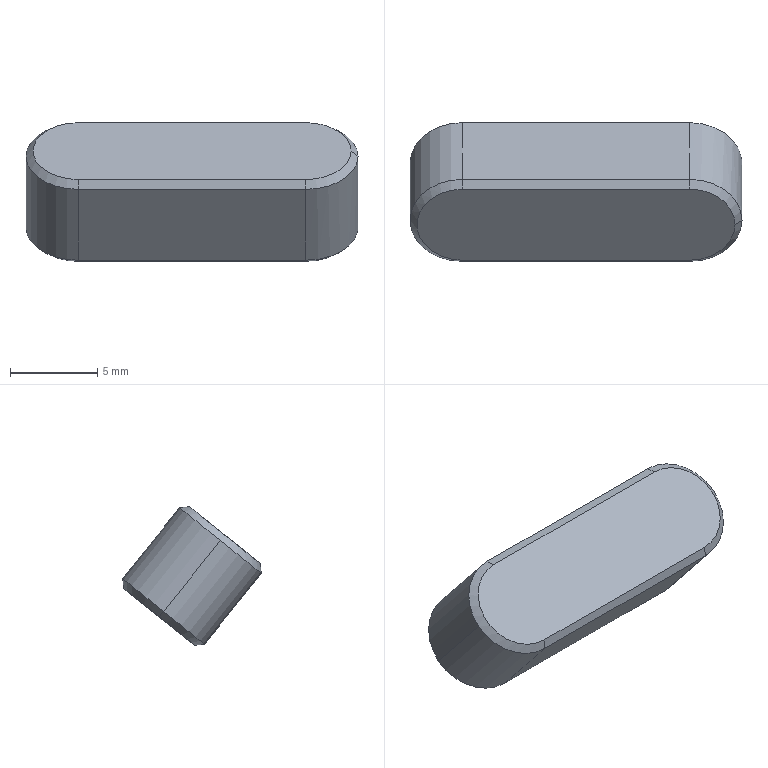Component | SolidWorks | Key6-6-25-2 | 1 solid | 17 faces | box 19 x 7.93 x 7.93 mm | volume 631 mm3 | plane 8 | cone 6 | cylinder 3 | commonest cylinder face diameters 6 x3
build123d program:
from build123d import *

# Parameters (mm, degrees)
BOSS_EXTRUDE1_DEPTH = 6
CHAMFER1_SIZE2      = 0.4
CHAMFER1_SIZE       = 0.4


with BuildPart() as part:
    # Sketch1 → Boss-Extrude1 (new body)
    with BuildSketch(Plane(origin=(0, 0, 4), x_dir=(1, 0, 0), z_dir=(0, -1, 0))):
        with BuildLine():
            Line((-3, 9), (-3, -4))
            ThreePointArc((-3, -4), (0, -7), (3, -4))
            Line((3, -4), (3, 9))
            ThreePointArc((3, 9), (0, 12), (-3, 9))
        make_face()
    extrude(amount=-BOSS_EXTRUDE1_DEPTH)

    # Chamfer1
    chamfer1_edges = [part.edges().sort_by_distance(p)[0] for p in [
        (0, 6, -3),
        (3, 6, 6.5),
        (0, 6, 16),
        (3, 0, 6.5),
        (0, 0, -3),
        (-3, 0, 6.5),
        (0, 0, 16),
        (-3, 6, 6.5),
    ]]
    chamfer(chamfer1_edges, length=CHAMFER1_SIZE, length2=CHAMFER1_SIZE2)


solid = part.part

# Placed as in the assembly
solid = solid.moved(Location((-531.299, 8.129, -10.145), (128.707, -90, 0)))
STEP:
#1=COLOUR_RGB('',0.7922,0.8196,0.9333);
#2=FILL_AREA_STYLE_COLOUR('',#1);
#3=FILL_AREA_STYLE('',(#2));
#4=SURFACE_STYLE_FILL_AREA(#3);
#5=SURFACE_SIDE_STYLE('',(#4));
#6=SURFACE_STYLE_USAGE(.BOTH.,#5);
#7=PRESENTATION_STYLE_ASSIGNMENT((#6));
#8=CARTESIAN_POINT('',(-21.531,0.3201,-0.3994));
#9=VERTEX_POINT('',#8);
#10=CARTESIAN_POINT('',(-21.429,0.3999,-0.3354));
#11=VERTEX_POINT('',#10);
#12=CARTESIAN_POINT('',(-21.429,0.3201,-0.3994));
#13=DIRECTION('',(-0.,0.6253,-0.7803));
#14=DIRECTION('',(-1.,-0.,-0.));
#15=AXIS2_PLACEMENT_3D('',#12,#13,#14);
#16=CIRCLE('',#15,0.1024);
#17=EDGE_CURVE('',#9,#11,#16,.T.);
#18=ORIENTED_EDGE('',*,*,#17,.F.);
#19=CARTESIAN_POINT('',(-21.547,0.3102,-0.3871));
#20=VERTEX_POINT('',#19);
#21=CARTESIAN_POINT('',(-21.547,0.3102,-0.3871));
#22=DIRECTION('',(-0.7071,-0.4422,0.5518));
#23=VECTOR('',#22,39.37);
#24=LINE('',#21,#23);
#25=EDGE_CURVE('',#9,#20,#24,.T.);
#26=ORIENTED_EDGE('',*,*,#25,.T.);
#27=CARTESIAN_POINT('',(-21.429,0.4024,-0.3132));
#28=VERTEX_POINT('',#27);
#29=CARTESIAN_POINT('',(-21.429,0.3102,-0.3871));
#30=DIRECTION('',(0.,-0.6253,0.7803));
#31=DIRECTION('',(-1.,-0.,-0.));
#32=AXIS2_PLACEMENT_3D('',#29,#30,#31);
#33=CIRCLE('',#32,0.1181);
#34=EDGE_CURVE('',#28,#20,#33,.T.);
#35=ORIENTED_EDGE('',*,*,#34,.F.);
#36=CARTESIAN_POINT('',(-21.429,0.3999,-0.3354));
#37=DIRECTION('',(-0.,0.1096,0.994));
#38=VECTOR('',#37,39.37);
#39=LINE('',#36,#38);
#40=EDGE_CURVE('',#11,#28,#39,.T.);
#41=ORIENTED_EDGE('',*,*,#40,.F.);
#42=EDGE_LOOP('',(#18,#26,#35,#41));
#43=FACE_OUTER_BOUND('',#42,.T.);
#44=CARTESIAN_POINT('',(-21.429,0.3102,-0.3871));
#45=DIRECTION('',(0.,-0.6253,0.7803));
#46=DIRECTION('',(-1.,-0.,-0.));
#47=AXIS2_PLACEMENT_3D('',#44,#45,#46);
#48=CONICAL_SURFACE('',#47,0.1181,0.7854);
#49=ADVANCED_FACE('',(#43),#48,.T.);
#50=CARTESIAN_POINT('',(-20.815,0.1723,-0.2151));
#51=VERTEX_POINT('',#50);
#52=CARTESIAN_POINT('',(-20.917,0.2522,-0.151));
#53=VERTEX_POINT('',#52);
#54=CARTESIAN_POINT('',(-20.917,0.1723,-0.2151));
#55=DIRECTION('',(0.,-0.6253,0.7803));
#56=DIRECTION('',(-1.,-0.,-0.));
#57=AXIS2_PLACEMENT_3D('',#54,#55,#56);
#58=CIRCLE('',#57,0.1024);
#59=EDGE_CURVE('',#51,#53,#58,.T.);
#60=ORIENTED_EDGE('',*,*,#59,.F.);
#61=CARTESIAN_POINT('',(-20.799,0.1822,-0.2273));
#62=VERTEX_POINT('',#61);
#63=CARTESIAN_POINT('',(-20.815,0.1723,-0.2151));
#64=DIRECTION('',(0.7071,0.4422,-0.5518));
#65=VECTOR('',#64,39.37);
#66=LINE('',#63,#65);
#67=EDGE_CURVE('',#51,#62,#66,.T.);
#68=ORIENTED_EDGE('',*,*,#67,.T.);
#69=CARTESIAN_POINT('',(-20.917,0.2744,-0.1535));
#70=VERTEX_POINT('',#69);
#71=CARTESIAN_POINT('',(-20.917,0.1822,-0.2273));
#72=DIRECTION('',(-0.,0.6253,-0.7803));
#73=DIRECTION('',(-1.,-0.,-0.));
#74=AXIS2_PLACEMENT_3D('',#71,#72,#73);
#75=CIRCLE('',#74,0.1181);
#76=EDGE_CURVE('',#70,#62,#75,.T.);
#77=ORIENTED_EDGE('',*,*,#76,.F.);
#78=CARTESIAN_POINT('',(-20.917,0.2744,-0.1535));
#79=DIRECTION('',(0.,-0.994,0.1096));
#80=VECTOR('',#79,39.37);
#81=LINE('',#78,#80);
#82=EDGE_CURVE('',#70,#53,#81,.T.);
#83=ORIENTED_EDGE('',*,*,#82,.T.);
#84=EDGE_LOOP('',(#60,#68,#77,#83));
#85=FACE_OUTER_BOUND('',#84,.T.);
#86=CARTESIAN_POINT('',(-20.917,0.1723,-0.2151));
#87=DIRECTION('',(-0.,0.6253,-0.7803));
#88=DIRECTION('',(1.,0.,0.));
#89=AXIS2_PLACEMENT_3D('',#86,#87,#88);
#90=CONICAL_SURFACE('',#89,0.1024,0.7854);
#91=ADVANCED_FACE('',(#85),#90,.T.);
#92=ORIENTED_EDGE('',*,*,#34,.T.);
#93=CARTESIAN_POINT('',(-21.547,0.1822,-0.2273));
#94=VERTEX_POINT('',#93);
#95=CARTESIAN_POINT('',(-21.547,0.3201,-0.3994));
#96=DIRECTION('',(0.,-0.6253,0.7803));
#97=VECTOR('',#96,39.37);
#98=LINE('',#95,#97);
#99=EDGE_CURVE('',#20,#94,#98,.T.);
#100=ORIENTED_EDGE('',*,*,#99,.T.);
#101=CARTESIAN_POINT('',(-21.429,0.2744,-0.1535));
#102=VERTEX_POINT('',#101);
#103=CARTESIAN_POINT('',(-21.429,0.1822,-0.2273));
#104=DIRECTION('',(-0.,0.6253,-0.7803));
#105=DIRECTION('',(-1.,-0.,-0.));
#106=AXIS2_PLACEMENT_3D('',#103,#104,#105);
#107=CIRCLE('',#106,0.1181);
#108=EDGE_CURVE('',#94,#102,#107,.T.);
#109=ORIENTED_EDGE('',*,*,#108,.T.);
#110=CARTESIAN_POINT('',(-21.429,0.4122,-0.3255));
#111=DIRECTION('',(0.,-0.6253,0.7803));
#112=VECTOR('',#111,39.37);
#113=LINE('',#110,#112);
#114=EDGE_CURVE('',#28,#102,#113,.T.);
#115=ORIENTED_EDGE('',*,*,#114,.F.);
#116=EDGE_LOOP('',(#92,#100,#109,#115));
#117=FACE_OUTER_BOUND('',#116,.T.);
#118=CARTESIAN_POINT('',(-21.429,0.3201,-0.3994));
#119=DIRECTION('',(0.,-0.6253,0.7803));
#120=DIRECTION('',(-1.,-0.,-0.));
#121=AXIS2_PLACEMENT_3D('',#118,#119,#120);
#122=CYLINDRICAL_SURFACE('',#121,0.1181);
#123=ADVANCED_FACE('',(#117),#122,.T.);
#124=CARTESIAN_POINT('',(-20.917,0.4024,-0.3132));
#125=VERTEX_POINT('',#124);
#126=CARTESIAN_POINT('',(-20.917,0.4122,-0.3255));
#127=DIRECTION('',(0.,-0.6253,0.7803));
#128=VECTOR('',#127,39.37);
#129=LINE('',#126,#128);
#130=EDGE_CURVE('',#125,#70,#129,.T.);
#131=ORIENTED_EDGE('',*,*,#130,.T.);
#132=ORIENTED_EDGE('',*,*,#76,.T.);
#133=CARTESIAN_POINT('',(-20.917,0.09002,-0.3012));
#134=VERTEX_POINT('',#133);
#135=CARTESIAN_POINT('',(-20.917,0.1822,-0.2273));
#136=DIRECTION('',(-0.,0.6253,-0.7803));
#137=DIRECTION('',(-1.,-0.,-0.));
#138=AXIS2_PLACEMENT_3D('',#135,#136,#137);
#139=CIRCLE('',#138,0.1181);
#140=EDGE_CURVE('',#62,#134,#139,.T.);
#141=ORIENTED_EDGE('',*,*,#140,.T.);
#142=CARTESIAN_POINT('',(-20.917,0.218,-0.461));
#143=VERTEX_POINT('',#142);
#144=CARTESIAN_POINT('',(-20.917,0.2279,-0.4733));
#145=DIRECTION('',(0.,-0.6253,0.7803));
#146=VECTOR('',#145,39.37);
#147=LINE('',#144,#146);
#148=EDGE_CURVE('',#143,#134,#147,.T.);
#149=ORIENTED_EDGE('',*,*,#148,.F.);
#150=CARTESIAN_POINT('',(-20.917,0.3102,-0.3871));
#151=DIRECTION('',(0.,-0.6253,0.7803));
#152=DIRECTION('',(-1.,-0.,-0.));
#153=AXIS2_PLACEMENT_3D('',#150,#151,#152);
#154=CIRCLE('',#153,0.1181);
#155=EDGE_CURVE('',#143,#125,#154,.T.);
#156=ORIENTED_EDGE('',*,*,#155,.T.);
#157=EDGE_LOOP('',(#131,#132,#141,#149,#156));
#158=FACE_OUTER_BOUND('',#157,.T.);
#159=CARTESIAN_POINT('',(-20.917,0.3201,-0.3994));
#160=DIRECTION('',(0.,-0.6253,0.7803));
#161=DIRECTION('',(-1.,-0.,-0.));
#162=AXIS2_PLACEMENT_3D('',#159,#160,#161);
#163=CYLINDRICAL_SURFACE('',#162,0.1181);
#164=ADVANCED_FACE('',(#158),#163,.T.);
#165=ORIENTED_EDGE('',*,*,#148,.T.);
#166=CARTESIAN_POINT('',(-21.429,0.09002,-0.3012));
#167=VERTEX_POINT('',#166);
#168=CARTESIAN_POINT('',(-21.429,0.09002,-0.3012));
#169=DIRECTION('',(-1.,-0.,-0.));
#170=VECTOR('',#169,39.37);
#171=LINE('',#168,#170);
#172=EDGE_CURVE('',#134,#167,#171,.T.);
#173=ORIENTED_EDGE('',*,*,#172,.T.);
#174=CARTESIAN_POINT('',(-21.429,0.218,-0.461));
#175=VERTEX_POINT('',#174);
#176=CARTESIAN_POINT('',(-21.429,0.2279,-0.4733));
#177=DIRECTION('',(0.,-0.6253,0.7803));
#178=VECTOR('',#177,39.37);
#179=LINE('',#176,#178);
#180=EDGE_CURVE('',#175,#167,#179,.T.);
#181=ORIENTED_EDGE('',*,*,#180,.F.);
#182=CARTESIAN_POINT('',(-20.917,0.218,-0.461));
#183=DIRECTION('',(1.,0.,0.));
#184=VECTOR('',#183,39.37);
#185=LINE('',#182,#184);
#186=EDGE_CURVE('',#175,#143,#185,.T.);
#187=ORIENTED_EDGE('',*,*,#186,.T.);
#188=EDGE_LOOP('',(#165,#173,#181,#187));
#189=FACE_OUTER_BOUND('',#188,.T.);
#190=CARTESIAN_POINT('',(-21.429,0.2279,-0.4733));
#191=DIRECTION('',(0.,-0.7803,-0.6253));
#192=DIRECTION('',(-1.,-0.,-0.));
#193=AXIS2_PLACEMENT_3D('',#190,#191,#192);
#194=PLANE('',#193);
#195=ADVANCED_FACE('',(#189),#194,.T.);
#196=ORIENTED_EDGE('',*,*,#99,.F.);
#197=CARTESIAN_POINT('',(-21.429,0.3102,-0.3871));
#198=DIRECTION('',(0.,-0.6253,0.7803));
#199=DIRECTION('',(-1.,-0.,-0.));
#200=AXIS2_PLACEMENT_3D('',#197,#198,#199);
#201=CIRCLE('',#200,0.1181);
#202=EDGE_CURVE('',#20,#175,#201,.T.);
#203=ORIENTED_EDGE('',*,*,#202,.T.);
#204=ORIENTED_EDGE('',*,*,#180,.T.);
#205=CARTESIAN_POINT('',(-21.429,0.1822,-0.2273));
#206=DIRECTION('',(-0.,0.6253,-0.7803));
#207=DIRECTION('',(-1.,0.,0.));
#208=AXIS2_PLACEMENT_3D('',#205,#206,#207);
#209=CIRCLE('',#208,0.1181);
#210=EDGE_CURVE('',#167,#94,#209,.T.);
#211=ORIENTED_EDGE('',*,*,#210,.T.);
#212=EDGE_LOOP('',(#196,#203,#204,#211));
#213=FACE_OUTER_BOUND('',#212,.T.);
#214=CARTESIAN_POINT('',(-21.429,0.3201,-0.3994));
#215=DIRECTION('',(0.,-0.6253,0.7803));
#216=DIRECTION('',(-1.,-0.,-0.));
#217=AXIS2_PLACEMENT_3D('',#214,#215,#216);
#218=CYLINDRICAL_SURFACE('',#217,0.1181);
#219=ADVANCED_FACE('',(#213),#218,.T.);
#220=ORIENTED_EDGE('',*,*,#114,.T.);
#221=CARTESIAN_POINT('',(-20.917,0.2744,-0.1535));
#222=DIRECTION('',(1.,0.,0.));
#223=VECTOR('',#222,39.37);
#224=LINE('',#221,#223);
#225=EDGE_CURVE('',#102,#70,#224,.T.);
#226=ORIENTED_EDGE('',*,*,#225,.T.);
#227=ORIENTED_EDGE('',*,*,#130,.F.);
#228=CARTESIAN_POINT('',(-21.429,0.4024,-0.3132));
#229=DIRECTION('',(-1.,-0.,-0.));
#230=VECTOR('',#229,39.37);
#231=LINE('',#228,#230);
#232=EDGE_CURVE('',#125,#28,#231,.T.);
#233=ORIENTED_EDGE('',*,*,#232,.T.);
#234=EDGE_LOOP('',(#220,#226,#227,#233));
#235=FACE_OUTER_BOUND('',#234,.T.);
#236=CARTESIAN_POINT('',(-20.917,0.4122,-0.3255));
#237=DIRECTION('',(-0.,0.7803,0.6253));
#238=DIRECTION('',(1.,0.,0.));
#239=AXIS2_PLACEMENT_3D('',#236,#237,#238);
#240=PLANE('',#239);
#241=ADVANCED_FACE('',(#235),#240,.T.);
#242=CARTESIAN_POINT('',(-21.429,0.2402,-0.4634));
#243=VERTEX_POINT('',#242);
#244=CARTESIAN_POINT('',(-21.429,0.3201,-0.3994));
#245=DIRECTION('',(-0.,0.6253,-0.7803));
#246=DIRECTION('',(-1.,0.,0.));
#247=AXIS2_PLACEMENT_3D('',#244,#245,#246);
#248=CIRCLE('',#247,0.1024);
#249=EDGE_CURVE('',#243,#9,#248,.T.);
#250=ORIENTED_EDGE('',*,*,#249,.T.);
#251=ORIENTED_EDGE('',*,*,#17,.T.);
#252=CARTESIAN_POINT('',(-20.917,0.3999,-0.3354));
#253=VERTEX_POINT('',#252);
#254=CARTESIAN_POINT('',(-20.917,0.3999,-0.3354));
#255=DIRECTION('',(1.,0.,0.));
#256=VECTOR('',#255,39.37);
#257=LINE('',#254,#256);
#258=EDGE_CURVE('',#11,#253,#257,.T.);
#259=ORIENTED_EDGE('',*,*,#258,.T.);
#260=CARTESIAN_POINT('',(-20.917,0.2402,-0.4634));
#261=VERTEX_POINT('',#260);
#262=CARTESIAN_POINT('',(-20.917,0.3201,-0.3994));
#263=DIRECTION('',(-0.,0.6253,-0.7803));
#264=DIRECTION('',(-1.,-0.,-0.));
#265=AXIS2_PLACEMENT_3D('',#262,#263,#264);
#266=CIRCLE('',#265,0.1024);
#267=EDGE_CURVE('',#253,#261,#266,.T.);
#268=ORIENTED_EDGE('',*,*,#267,.T.);
#269=CARTESIAN_POINT('',(-21.429,0.2402,-0.4634));
#270=DIRECTION('',(-1.,-0.,-0.));
#271=VECTOR('',#270,39.37);
#272=LINE('',#269,#271);
#273=EDGE_CURVE('',#261,#243,#272,.T.);
#274=ORIENTED_EDGE('',*,*,#273,.T.);
#275=EDGE_LOOP('',(#250,#251,#259,#268,#274));
#276=FACE_OUTER_BOUND('',#275,.T.);
#277=CARTESIAN_POINT('',(-20.917,0.3201,-0.3994));
#278=DIRECTION('',(0.,-0.6253,0.7803));
#279=DIRECTION('',(-1.,-0.,-0.));
#280=AXIS2_PLACEMENT_3D('',#277,#278,#279);
#281=PLANE('',#280);
#282=ADVANCED_FACE('',(#276),#281,.F.);
#283=CARTESIAN_POINT('',(-21.429,0.2522,-0.151));
#284=VERTEX_POINT('',#283);
#285=CARTESIAN_POINT('',(-21.429,0.09246,-0.2791));
#286=VERTEX_POINT('',#285);
#287=CARTESIAN_POINT('',(-21.429,0.1723,-0.2151));
#288=DIRECTION('',(0.,-0.6253,0.7803));
#289=DIRECTION('',(-1.,-0.,-0.));
#290=AXIS2_PLACEMENT_3D('',#287,#288,#289);
#291=CIRCLE('',#290,0.1024);
#292=EDGE_CURVE('',#284,#286,#291,.T.);
#293=ORIENTED_EDGE('',*,*,#292,.T.);
#294=CARTESIAN_POINT('',(-20.917,0.09246,-0.2791));
#295=VERTEX_POINT('',#294);
#296=CARTESIAN_POINT('',(-20.917,0.09246,-0.2791));
#297=DIRECTION('',(1.,0.,0.));
#298=VECTOR('',#297,39.37);
#299=LINE('',#296,#298);
#300=EDGE_CURVE('',#286,#295,#299,.T.);
#301=ORIENTED_EDGE('',*,*,#300,.T.);
#302=CARTESIAN_POINT('',(-20.917,0.1723,-0.2151));
#303=DIRECTION('',(0.,-0.6253,0.7803));
#304=DIRECTION('',(-1.,-0.,-0.));
#305=AXIS2_PLACEMENT_3D('',#302,#303,#304);
#306=CIRCLE('',#305,0.1024);
#307=EDGE_CURVE('',#295,#51,#306,.T.);
#308=ORIENTED_EDGE('',*,*,#307,.T.);
#309=ORIENTED_EDGE('',*,*,#59,.T.);
#310=CARTESIAN_POINT('',(-20.917,0.2522,-0.151));
#311=DIRECTION('',(-1.,-0.,-0.));
#312=VECTOR('',#311,39.37);
#313=LINE('',#310,#312);
#314=EDGE_CURVE('',#53,#284,#313,.T.);
#315=ORIENTED_EDGE('',*,*,#314,.T.);
#316=EDGE_LOOP('',(#293,#301,#308,#309,#315));
#317=FACE_OUTER_BOUND('',#316,.T.);
#318=CARTESIAN_POINT('',(-20.917,0.1723,-0.2151));
#319=DIRECTION('',(0.,-0.6253,0.7803));
#320=DIRECTION('',(-1.,-0.,-0.));
#321=AXIS2_PLACEMENT_3D('',#318,#319,#320);
#322=PLANE('',#321);
#323=ADVANCED_FACE('',(#317),#322,.T.);
#324=ORIENTED_EDGE('',*,*,#82,.F.);
#325=ORIENTED_EDGE('',*,*,#225,.F.);
#326=CARTESIAN_POINT('',(-21.429,0.2522,-0.151));
#327=DIRECTION('',(-0.,0.994,-0.1096));
#328=VECTOR('',#327,39.37);
#329=LINE('',#326,#328);
#330=EDGE_CURVE('',#284,#102,#329,.T.);
#331=ORIENTED_EDGE('',*,*,#330,.F.);
#332=ORIENTED_EDGE('',*,*,#314,.F.);
#333=EDGE_LOOP('',(#324,#325,#331,#332));
#334=FACE_OUTER_BOUND('',#333,.T.);
#335=CARTESIAN_POINT('',(-20.917,0.2522,-0.151));
#336=DIRECTION('',(0.,-0.1096,-0.994));
#337=DIRECTION('',(-1.,-0.,-0.));
#338=AXIS2_PLACEMENT_3D('',#335,#336,#337);
#339=PLANE('',#338);
#340=ADVANCED_FACE('',(#334),#339,.F.);
#341=ORIENTED_EDGE('',*,*,#330,.T.);
#342=ORIENTED_EDGE('',*,*,#108,.F.);
#343=ORIENTED_EDGE('',*,*,#210,.F.);
#344=CARTESIAN_POINT('',(-21.429,0.09246,-0.2791));
#345=DIRECTION('',(0.,-0.1096,-0.994));
#346=VECTOR('',#345,39.37);
#347=LINE('',#344,#346);
#348=EDGE_CURVE('',#286,#167,#347,.T.);
#349=ORIENTED_EDGE('',*,*,#348,.F.);
#350=ORIENTED_EDGE('',*,*,#292,.F.);
#351=EDGE_LOOP('',(#341,#342,#343,#349,#350));
#352=FACE_OUTER_BOUND('',#351,.T.);
#353=CARTESIAN_POINT('',(-21.429,0.1723,-0.2151));
#354=DIRECTION('',(-0.,0.6253,-0.7803));
#355=DIRECTION('',(1.,0.,0.));
#356=AXIS2_PLACEMENT_3D('',#353,#354,#355);
#357=CONICAL_SURFACE('',#356,0.1024,0.7854);
#358=ADVANCED_FACE('',(#352),#357,.T.);
#359=ORIENTED_EDGE('',*,*,#67,.F.);
#360=ORIENTED_EDGE('',*,*,#307,.F.);
#361=CARTESIAN_POINT('',(-20.917,0.09002,-0.3012));
#362=DIRECTION('',(-0.,0.1096,0.994));
#363=VECTOR('',#362,39.37);
#364=LINE('',#361,#363);
#365=EDGE_CURVE('',#134,#295,#364,.T.);
#366=ORIENTED_EDGE('',*,*,#365,.F.);
#367=ORIENTED_EDGE('',*,*,#140,.F.);
#368=EDGE_LOOP('',(#359,#360,#366,#367));
#369=FACE_OUTER_BOUND('',#368,.T.);
#370=CARTESIAN_POINT('',(-20.917,0.1723,-0.2151));
#371=DIRECTION('',(-0.,0.6253,-0.7803));
#372=DIRECTION('',(1.,0.,0.));
#373=AXIS2_PLACEMENT_3D('',#370,#371,#372);
#374=CONICAL_SURFACE('',#373,0.1024,0.7854);
#375=ADVANCED_FACE('',(#369),#374,.T.);
#376=ORIENTED_EDGE('',*,*,#348,.T.);
#377=ORIENTED_EDGE('',*,*,#172,.F.);
#378=ORIENTED_EDGE('',*,*,#365,.T.);
#379=ORIENTED_EDGE('',*,*,#300,.F.);
#380=EDGE_LOOP('',(#376,#377,#378,#379));
#381=FACE_OUTER_BOUND('',#380,.T.);
#382=CARTESIAN_POINT('',(-20.917,0.09246,-0.2791));
#383=DIRECTION('',(-0.,0.994,-0.1096));
#384=DIRECTION('',(1.,0.,0.));
#385=AXIS2_PLACEMENT_3D('',#382,#383,#384);
#386=PLANE('',#385);
#387=ADVANCED_FACE('',(#381),#386,.F.);
#388=CARTESIAN_POINT('',(-21.429,0.2402,-0.4634));
#389=DIRECTION('',(0.,-0.994,0.1096));
#390=VECTOR('',#389,39.37);
#391=LINE('',#388,#390);
#392=EDGE_CURVE('',#243,#175,#391,.T.);
#393=ORIENTED_EDGE('',*,*,#392,.F.);
#394=ORIENTED_EDGE('',*,*,#273,.F.);
#395=CARTESIAN_POINT('',(-20.917,0.218,-0.461));
#396=DIRECTION('',(-0.,0.994,-0.1096));
#397=VECTOR('',#396,39.37);
#398=LINE('',#395,#397);
#399=EDGE_CURVE('',#143,#261,#398,.T.);
#400=ORIENTED_EDGE('',*,*,#399,.F.);
#401=ORIENTED_EDGE('',*,*,#186,.F.);
#402=EDGE_LOOP('',(#393,#394,#400,#401));
#403=FACE_OUTER_BOUND('',#402,.T.);
#404=CARTESIAN_POINT('',(-21.429,0.218,-0.461));
#405=DIRECTION('',(0.,-0.1096,-0.994));
#406=DIRECTION('',(-1.,-0.,-0.));
#407=AXIS2_PLACEMENT_3D('',#404,#405,#406);
#408=PLANE('',#407);
#409=ADVANCED_FACE('',(#403),#408,.T.);
#410=ORIENTED_EDGE('',*,*,#399,.T.);
#411=ORIENTED_EDGE('',*,*,#267,.F.);
#412=CARTESIAN_POINT('',(-20.917,0.4024,-0.3132));
#413=DIRECTION('',(0.,-0.1096,-0.994));
#414=VECTOR('',#413,39.37);
#415=LINE('',#412,#414);
#416=EDGE_CURVE('',#125,#253,#415,.T.);
#417=ORIENTED_EDGE('',*,*,#416,.F.);
#418=ORIENTED_EDGE('',*,*,#155,.F.);
#419=EDGE_LOOP('',(#410,#411,#417,#418));
#420=FACE_OUTER_BOUND('',#419,.T.);
#421=CARTESIAN_POINT('',(-20.917,0.3102,-0.3871));
#422=DIRECTION('',(0.,-0.6253,0.7803));
#423=DIRECTION('',(-1.,-0.,-0.));
#424=AXIS2_PLACEMENT_3D('',#421,#422,#423);
#425=CONICAL_SURFACE('',#424,0.1181,0.7854);
#426=ADVANCED_FACE('',(#420),#425,.T.);
#427=ORIENTED_EDGE('',*,*,#25,.F.);
#428=ORIENTED_EDGE('',*,*,#249,.F.);
#429=ORIENTED_EDGE('',*,*,#392,.T.);
#430=ORIENTED_EDGE('',*,*,#202,.F.);
#431=EDGE_LOOP('',(#427,#428,#429,#430));
#432=FACE_OUTER_BOUND('',#431,.T.);
#433=CARTESIAN_POINT('',(-21.429,0.3102,-0.3871));
#434=DIRECTION('',(0.,-0.6253,0.7803));
#435=DIRECTION('',(-1.,-0.,-0.));
#436=AXIS2_PLACEMENT_3D('',#433,#434,#435);
#437=CONICAL_SURFACE('',#436,0.1181,0.7854);
#438=ADVANCED_FACE('',(#432),#437,.T.);
#439=ORIENTED_EDGE('',*,*,#416,.T.);
#440=ORIENTED_EDGE('',*,*,#258,.F.);
#441=ORIENTED_EDGE('',*,*,#40,.T.);
#442=ORIENTED_EDGE('',*,*,#232,.F.);
#443=EDGE_LOOP('',(#439,#440,#441,#442));
#444=FACE_OUTER_BOUND('',#443,.T.);
#445=CARTESIAN_POINT('',(-20.917,0.4024,-0.3132));
#446=DIRECTION('',(-0.,0.994,-0.1096));
#447=DIRECTION('',(1.,0.,0.));
#448=AXIS2_PLACEMENT_3D('',#445,#446,#447);
#449=PLANE('',#448);
#450=ADVANCED_FACE('',(#444),#449,.T.);
#451=CLOSED_SHELL('',(#49,#91,#123,#164,#195,#219,#241,#282,#323,#340,#358,#375,#387,#409,#426,#438,#450));
#452=MANIFOLD_SOLID_BREP('',#451);
#453=STYLED_ITEM('',(#7),#452);
#454=PRESENTATION_LAYER_ASSIGNMENT('','',(#453));
#455=CARTESIAN_POINT('',(0.,0.,0.));
#456=DIRECTION('',(0.,0.,1.));
#457=DIRECTION('',(1.,0.,0.));
#458=AXIS2_PLACEMENT_3D('',#455,#456,#457);
#459=(LENGTH_UNIT()NAMED_UNIT(*)SI_UNIT($,.METRE.));
#460=LENGTH_MEASURE_WITH_UNIT(LENGTH_MEASURE(0.0254),#459);
#461=DIMENSIONAL_EXPONENTS(1.,0.,0.,0.,0.,0.,0.);
#462=(CONVERSION_BASED_UNIT('',#460)LENGTH_UNIT()NAMED_UNIT(#461));
#463=UNCERTAINTY_MEASURE_WITH_UNIT(LENGTH_MEASURE(0.00001),#462,'','');
#464=(NAMED_UNIT(*)PLANE_ANGLE_UNIT()SI_UNIT($,.RADIAN.));
#465=(NAMED_UNIT(*)SI_UNIT($,.STERADIAN.)SOLID_ANGLE_UNIT());
#466=(GEOMETRIC_REPRESENTATION_CONTEXT(3)GLOBAL_UNCERTAINTY_ASSIGNED_CONTEXT((#463))GLOBAL_UNIT_ASSIGNED_CONTEXT((#462,#464,#465))REPRESENTATION_CONTEXT('',''));
#467=ADVANCED_BREP_SHAPE_REPRESENTATION('',(#452,#458),#466);
#468=(LENGTH_UNIT()NAMED_UNIT(*)SI_UNIT($,.METRE.));
#469=LENGTH_MEASURE_WITH_UNIT(LENGTH_MEASURE(0.0254),#468);
#470=DIMENSIONAL_EXPONENTS(1.,0.,0.,0.,0.,0.,0.);
#471=(CONVERSION_BASED_UNIT('',#469)LENGTH_UNIT()NAMED_UNIT(#470));
#472=UNCERTAINTY_MEASURE_WITH_UNIT(LENGTH_MEASURE(0.00001),#471,'','');
#473=(NAMED_UNIT(*)PLANE_ANGLE_UNIT()SI_UNIT($,.RADIAN.));
#474=(NAMED_UNIT(*)SI_UNIT($,.STERADIAN.)SOLID_ANGLE_UNIT());
#475=(GEOMETRIC_REPRESENTATION_CONTEXT(3)GLOBAL_UNCERTAINTY_ASSIGNED_CONTEXT((#472))GLOBAL_UNIT_ASSIGNED_CONTEXT((#471,#473,#474))REPRESENTATION_CONTEXT('',''));
#476=MECHANICAL_DESIGN_GEOMETRIC_PRESENTATION_REPRESENTATION('',(#453),#475);